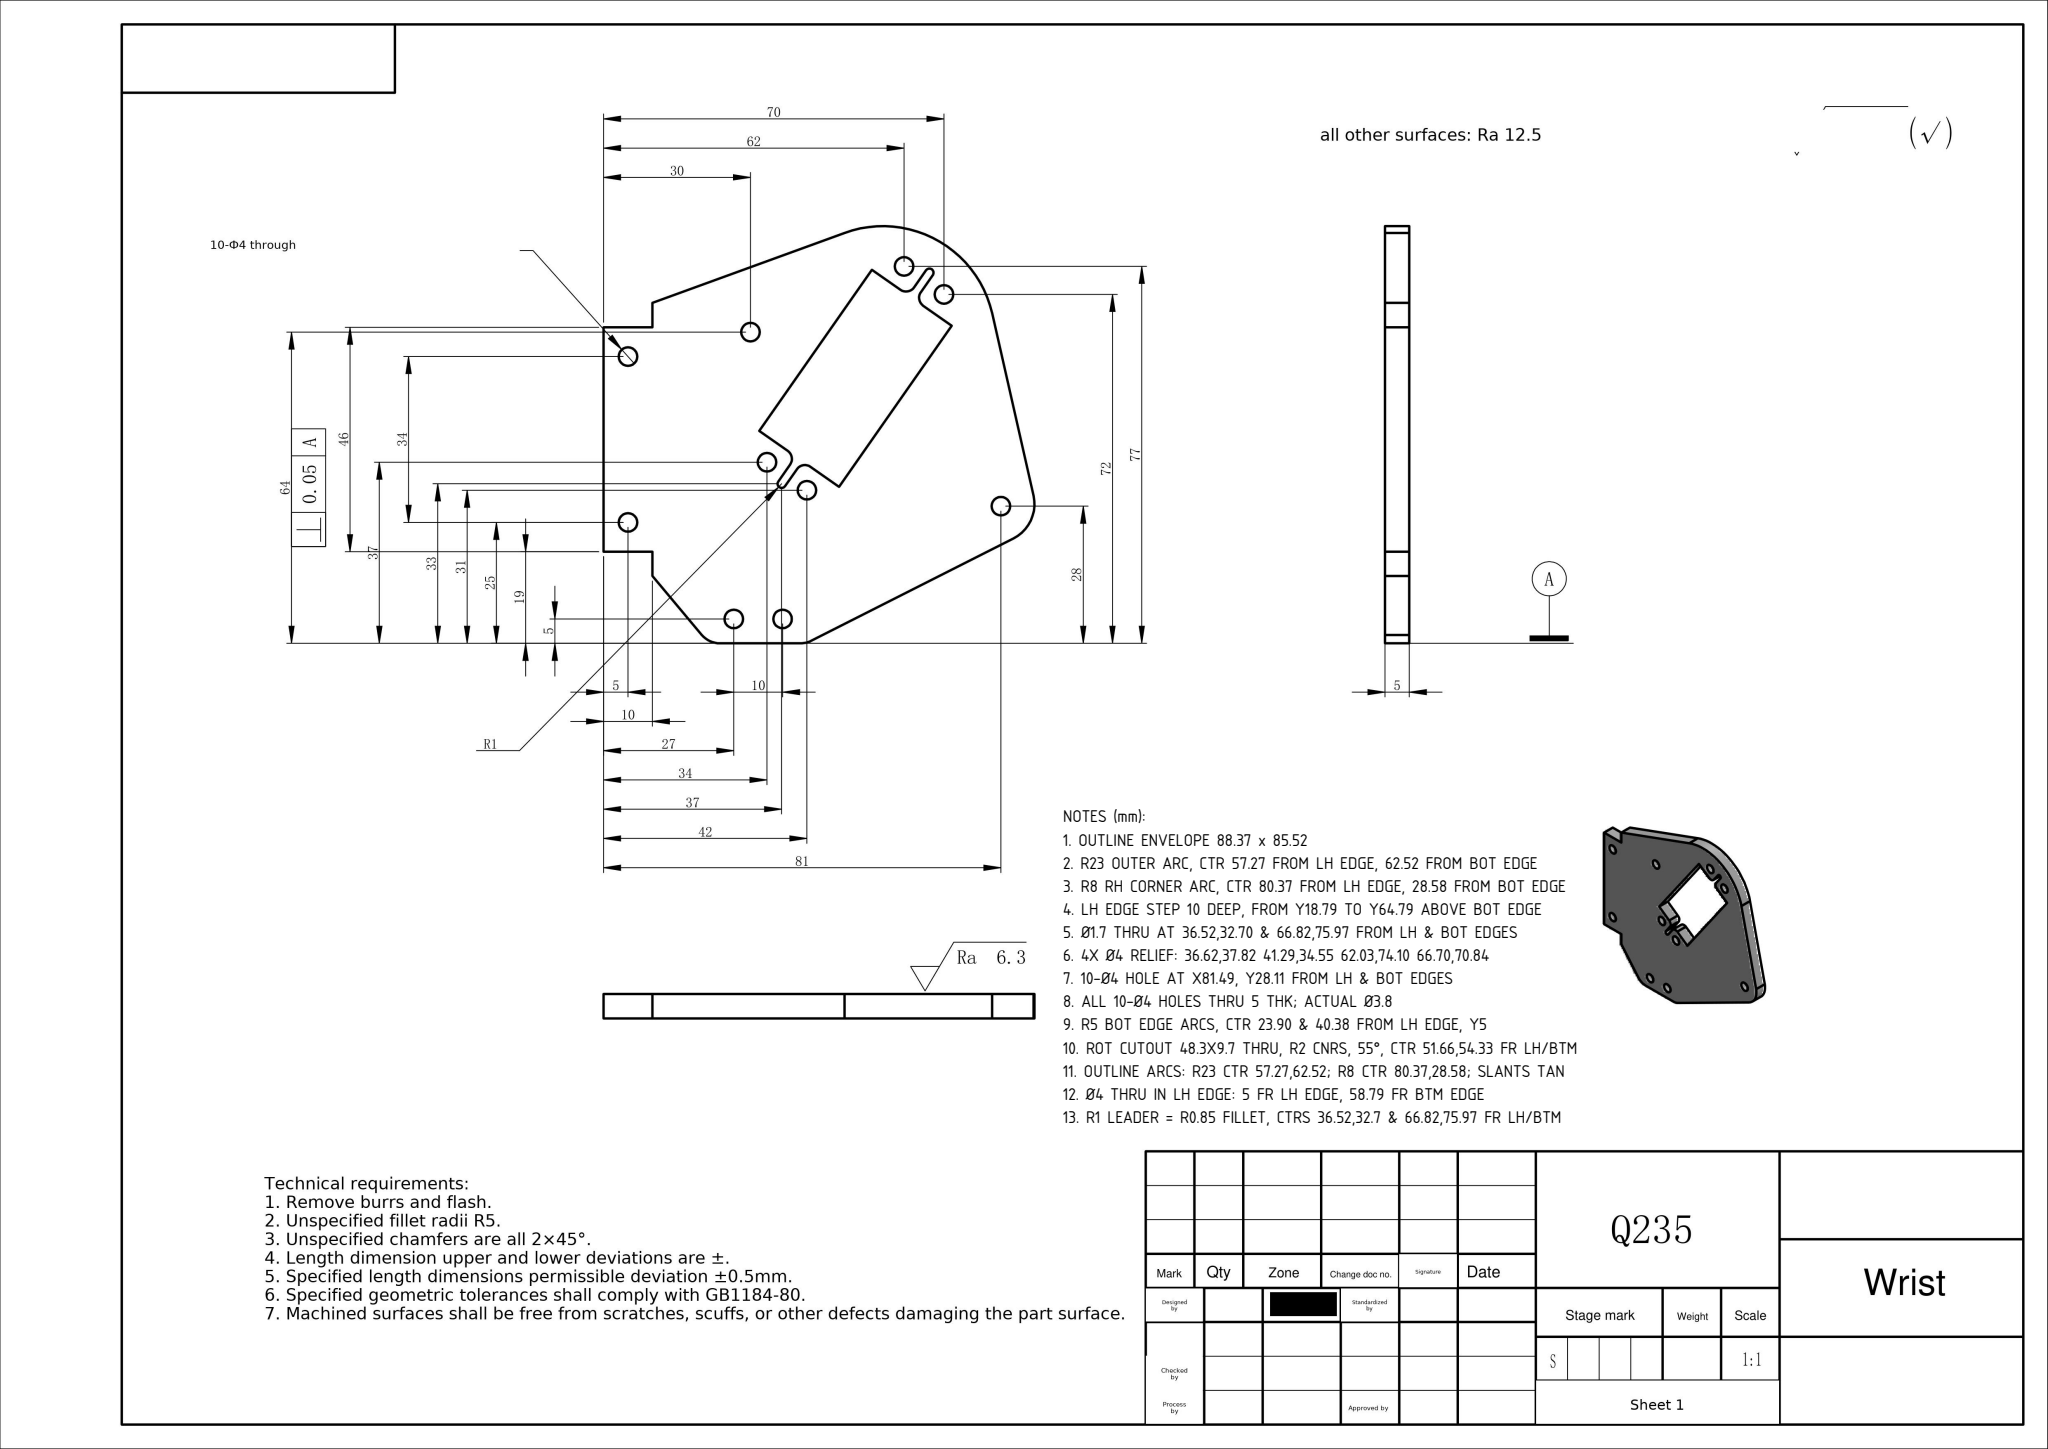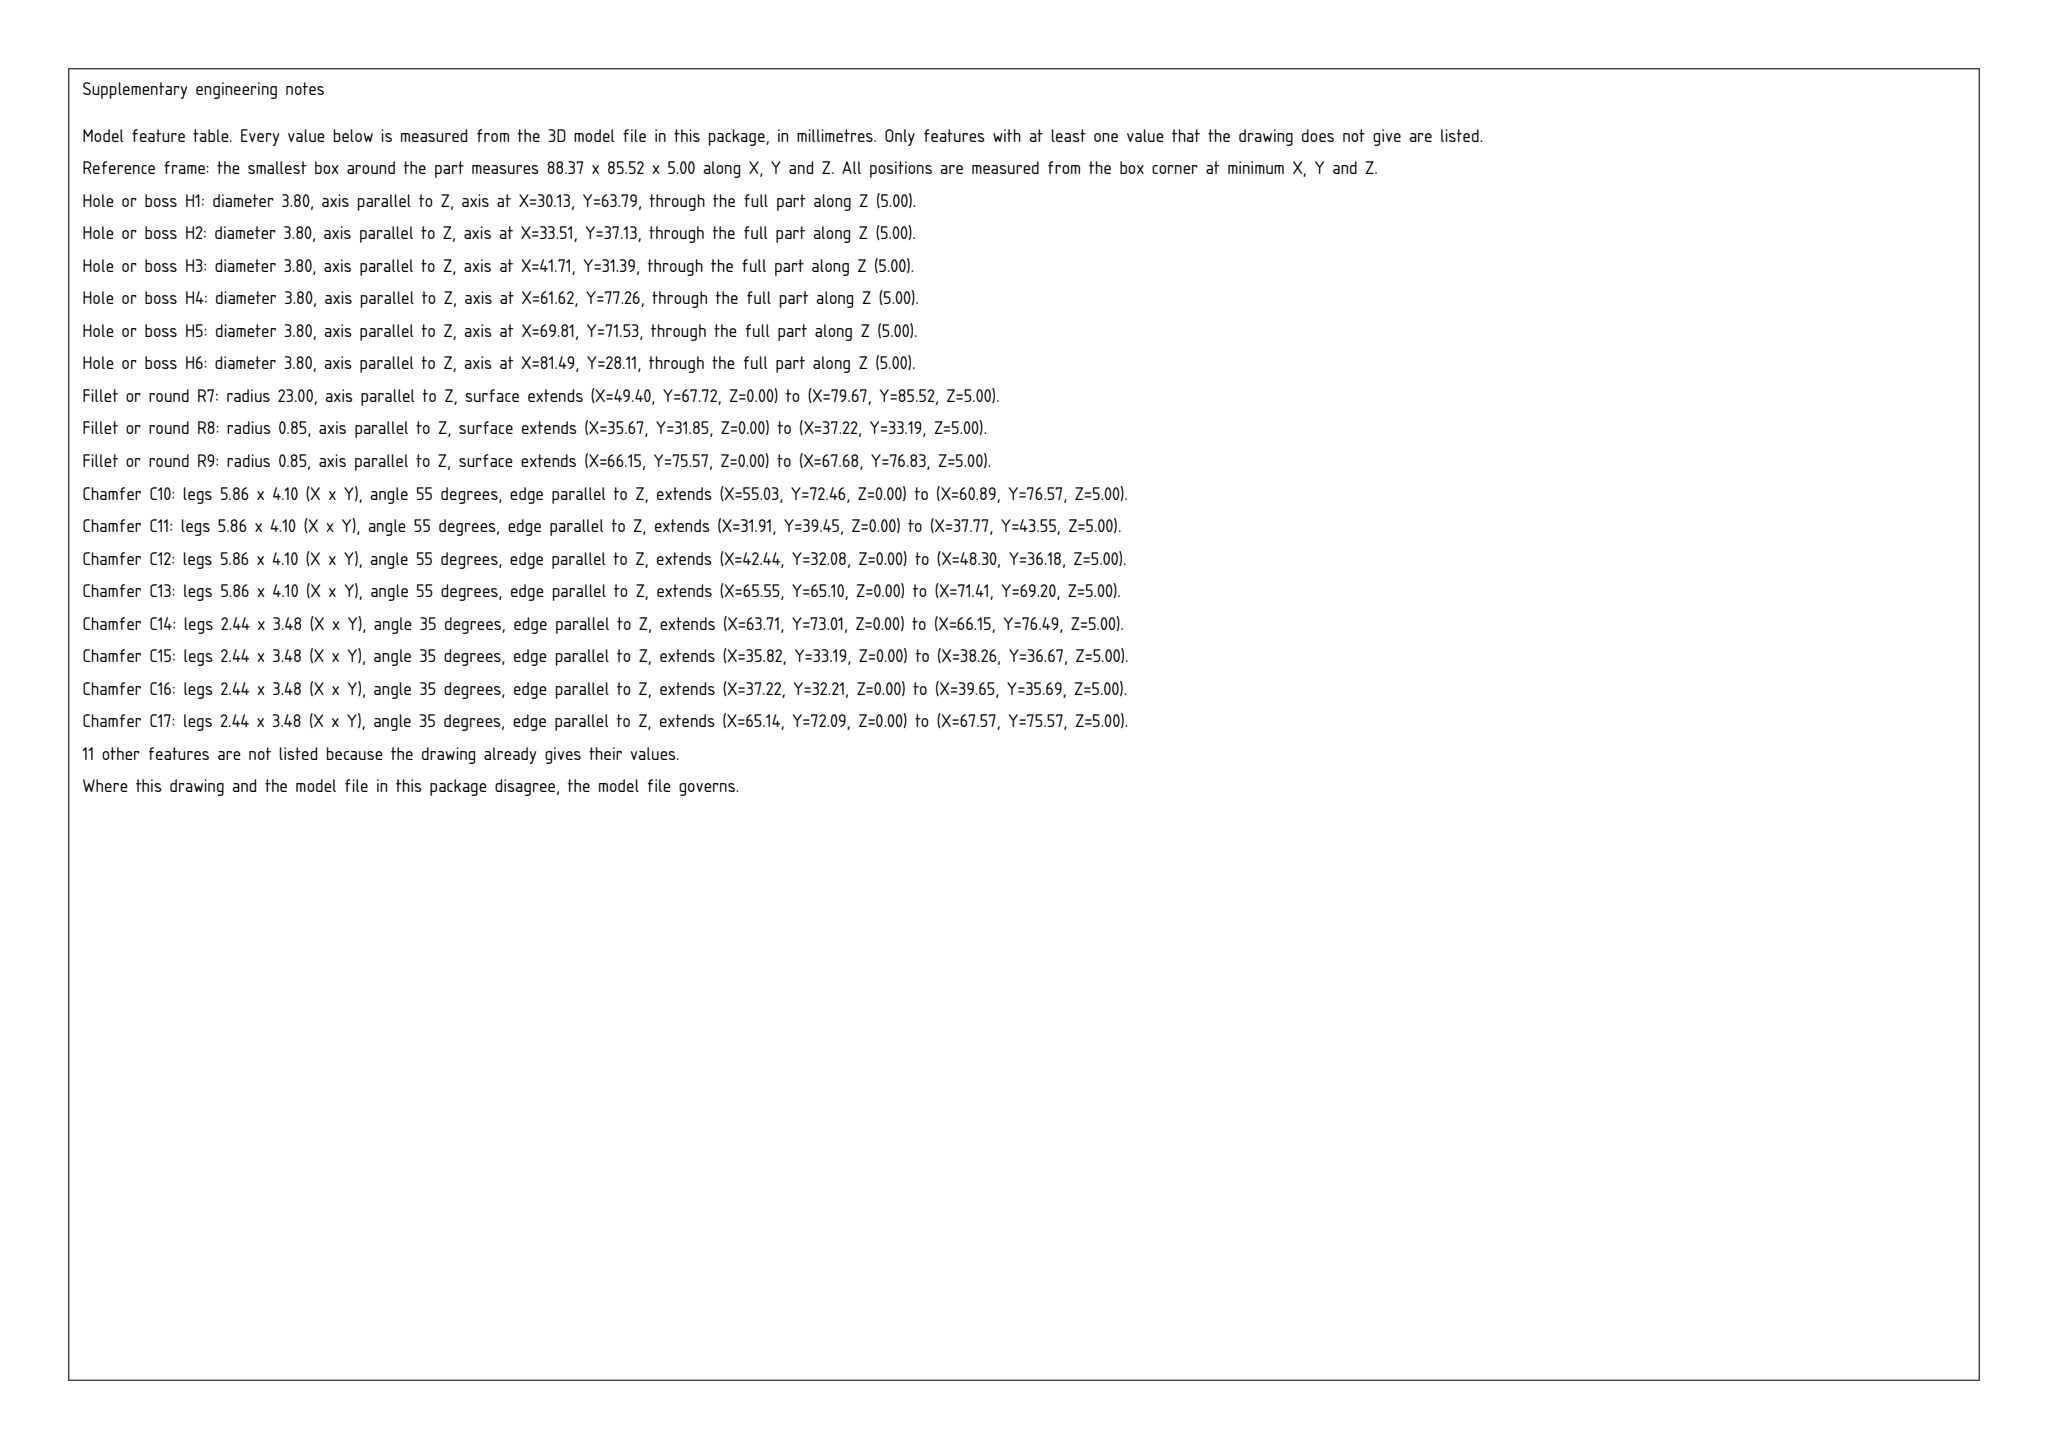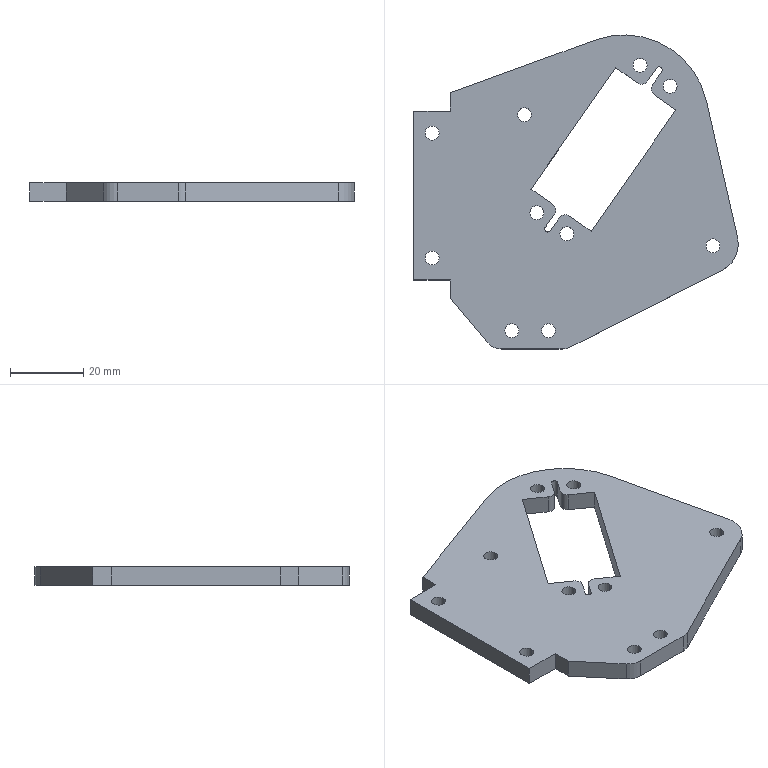Part | SolidWorks | mm | 1 solid | 54 faces | box 88.37 x 85.52 x 5 mm | volume 24067 mm3 | cylinder 32 | plane 22 | commonest cylinder face diameters 3.8 x20 4 x5 1.7 x2 10 x2 16 x1 46 x1 1.706 x1
Drawing notes:
OUTLINE ENVELOPE 88.37 x 85.52 | from the solid: bbox_xyz [88.37, 85.516, 5.0]
R23 OUTER ARC, CTR 57.27 FROM LH EDGE, 62.52 FROM BOT EDGE | from the solid: cylinder dia 46, axis z, pos [57.27, 62.52]
R8 RH CORNER ARC, CTR 80.37 FROM LH EDGE, 28.58 FROM BOT EDGE | from the solid: cylinder dia 16, axis z, pos [80.37, 28.58]
LH EDGE STEP 10 DEEP, FROM Y18.79 TO Y64.79 ABOVE BOT EDGE | from the solid: planes x=0, x=10 (2), y=18.79, y=64.79
Ø1.7 THRU AT 36.52,32.70 & 66.82,75.97 FROM LH & BOT EDGES | from the solid: cylinders dia 1.7 [36.52,32.7] and 1.706 [66.82,75.97], L=5
4X Ø4 RELIEF: 36.62,37.82 41.29,34.55 62.03,74.10 66.70,70.84 | from the solid: cylinders dia 4.0, axis z, 4 positions, length 5.0 thru
10-Ø4 HOLE AT X81.49, Y28.11 FROM LH & BOT EDGES | from the solid: cylinder dia 3.8 at [81.49, 28.11], thru 5.0
ALL 10-Ø4 HOLES THRU 5 THK; ACTUAL Ø3.8 | from the solid: 10 cylinders dia 3.8, axis z, length 5.0
R5 BOT EDGE ARCS, CTR 23.90 & 40.38 FROM LH EDGE, Y5 | from the solid: cylinders dia 10 at [23.9,5.0] and [40.38,5.0], L=5
ROT CUTOUT 48.3X9.7 THRU, R2 CNRS, 55°, CTR 51.66,54.33 FR LH/BTM | from the solid: 4X Ø4.0 z-cyl corner arcs at (36.62,37.82),(41.29,34.55),(62.03,74.1),(66.7,70.84): 44.30 x 5.70 ctr-to-ctr => 48.3 x 9.7 w/ R2 corners, long axis atan(36.28/25.41)=55.0 deg, ctr (51.66,54.33)
OUTLINE ARCS: R23 CTR 57.27,62.52; R8 CTR 80.37,28.58; SLANTS TAN | from the solid: Ø46 z-cyl at (57.27,62.52) => R23, tangent to y=85.52 top of bbox; Ø16 z-cyl at (80.37,28.58) => R8, tangent to x=88.37 bbox max
Ø4 THRU IN LH EDGE: 5 FR LH EDGE, 58.79 FR BTM EDGE | from the solid: Ø3.8 (Ø4 callout) z-cyl at (5.0,58.79), length 5.0, one of the 10-Ø4 through holes
R1 LEADER = R0.85 FILLET, CTRS 36.52,32.7 & 66.82,75.97 FR LH/BTM | from the solid: Ø1.7 z-cyl at (36.52,32.7) and Ø1.706 z-cyl at (66.82,75.97), length 5.0 => R0.85 fillets
build123d program:
from build123d import *

# Parameters (mm, degrees)
ESQUISSE1_R        = 1.9
BOSS_EXTRU_1_DEPTH = 5


with BuildPart() as part:
    # Esquisse1 → Boss.-Extru.1 (new body)
    with BuildSketch(Plane.XY):
        with BuildLine():
            Line((40.548, -21.276), (-0.9757, -42.265))
            ThreePointArc((-0.9757, -42.265), (-2.031, -42.633), (-3.142, -42.758))
            Line((-3.142, -42.758), (-19.618, -42.758))
            ThreePointArc((-19.618, -42.758), (-21.686, -42.311), (-23.383, -41.048))
            Line((-23.383, -41.048), (-33.52, -28.968))
            Line((-33.52, -28.968), (-33.52, -23.969))
            Line((-33.52, -23.969), (-43.52, -23.969))
            Line((-43.52, -23.969), (-43.52, 22.031))
            Line((-43.52, 22.031), (-33.52, 22.031))
            Line((-33.52, 22.031), (-33.52, 27.031))
            Line((-33.52, 27.031), (5.88, 41.371))
            ThreePointArc((5.88, 41.371), (24.71, 39.977), (36.152, 24.957))
            Line((36.152, 24.957), (44.673, -12.505))
            ThreePointArc((44.673, -12.505), (44.09, -17.587), (40.548, -21.276))
        make_face()
        with Locations((37.969, -14.646)):
            Circle(ESQUISSE1_R, mode=Mode.SUBTRACT)
        with Locations((26.291, 28.768)):
            Circle(ESQUISSE1_R, mode=Mode.SUBTRACT)
        with Locations((18.099, 34.504)):
            Circle(ESQUISSE1_R, mode=Mode.SUBTRACT)
        with Locations((-1.814, -11.37)):
            Circle(ESQUISSE1_R, mode=Mode.SUBTRACT)
        with Locations((-10.006, -5.635)):
            Circle(ESQUISSE1_R, mode=Mode.SUBTRACT)
        with Locations((-13.389, 21.031)):
            Circle(ESQUISSE1_R, mode=Mode.SUBTRACT)
        with Locations((-6.818, -37.758)):
            Circle(ESQUISSE1_R, mode=Mode.SUBTRACT)
        with Locations((-16.818, -37.758)):
            Circle(ESQUISSE1_R, mode=Mode.SUBTRACT)
        with Locations((-38.52, -17.969)):
            Circle(ESQUISSE1_R, mode=Mode.SUBTRACT)
        with Locations((-38.52, 16.031)):
            Circle(ESQUISSE1_R, mode=Mode.SUBTRACT)
        with BuildLine():
            Line((21.617, 29.329), (24.055, 32.81))
            ThreePointArc((24.055, 32.81), (23.767, 33.932), (22.625, 33.732))
            Line((22.625, 33.732), (20.188, 30.251))
            ThreePointArc((20.188, 30.251), (18.892, 29.381), (17.366, 29.707))
            Line((17.366, 29.707), (11.509, 33.808))
            Line((11.509, 33.808), (-11.607, 0.7965))
            Line((-11.607, 0.7965), (-5.75, -3.305))
            ThreePointArc((-5.75, -3.305), (-4.927, -4.596), (-5.258, -6.09))
            Line((-5.258, -6.09), (-7.696, -9.571))
            ThreePointArc((-7.696, -9.571), (-7.487, -10.755), (-6.304, -10.546))
            Line((-6.304, -10.546), (-3.866, -7.065))
            ThreePointArc((-3.866, -7.065), (-2.575, -6.243), (-1.08, -6.574))
            Line((-1.08, -6.574), (4.776, -10.675))
            Line((4.776, -10.675), (27.892, 22.337))
            Line((27.892, 22.337), (22.031, 26.44))
            ThreePointArc((22.031, 26.44), (21.199, 27.795), (21.617, 29.329))
        make_face(mode=Mode.SUBTRACT)
    extrude(amount=BOSS_EXTRU_1_DEPTH)


solid = part.part